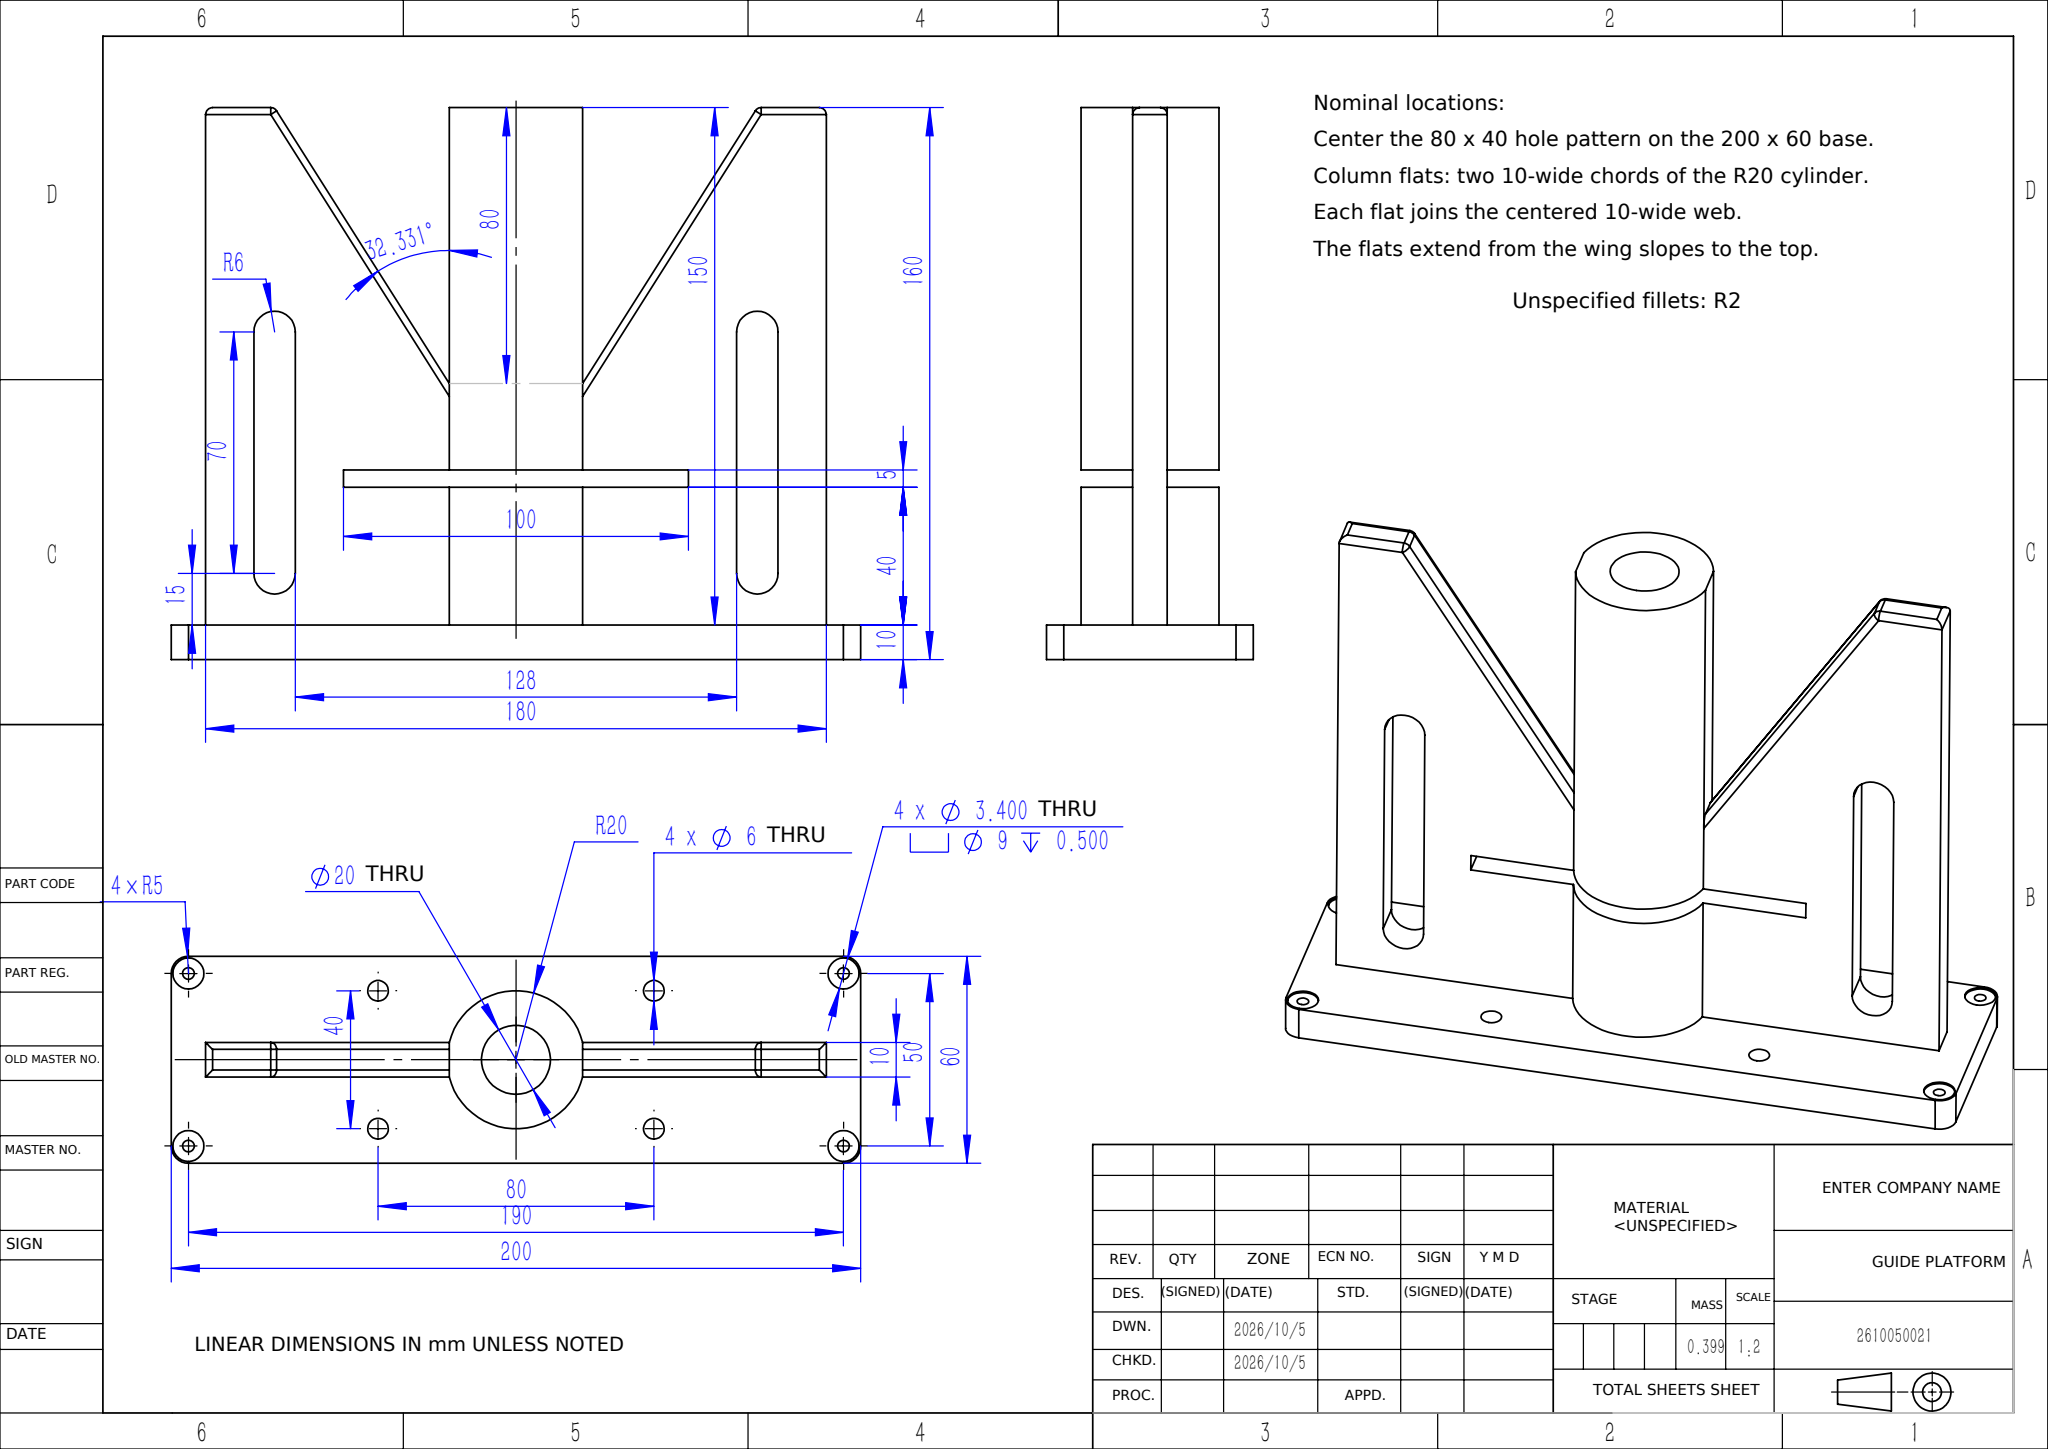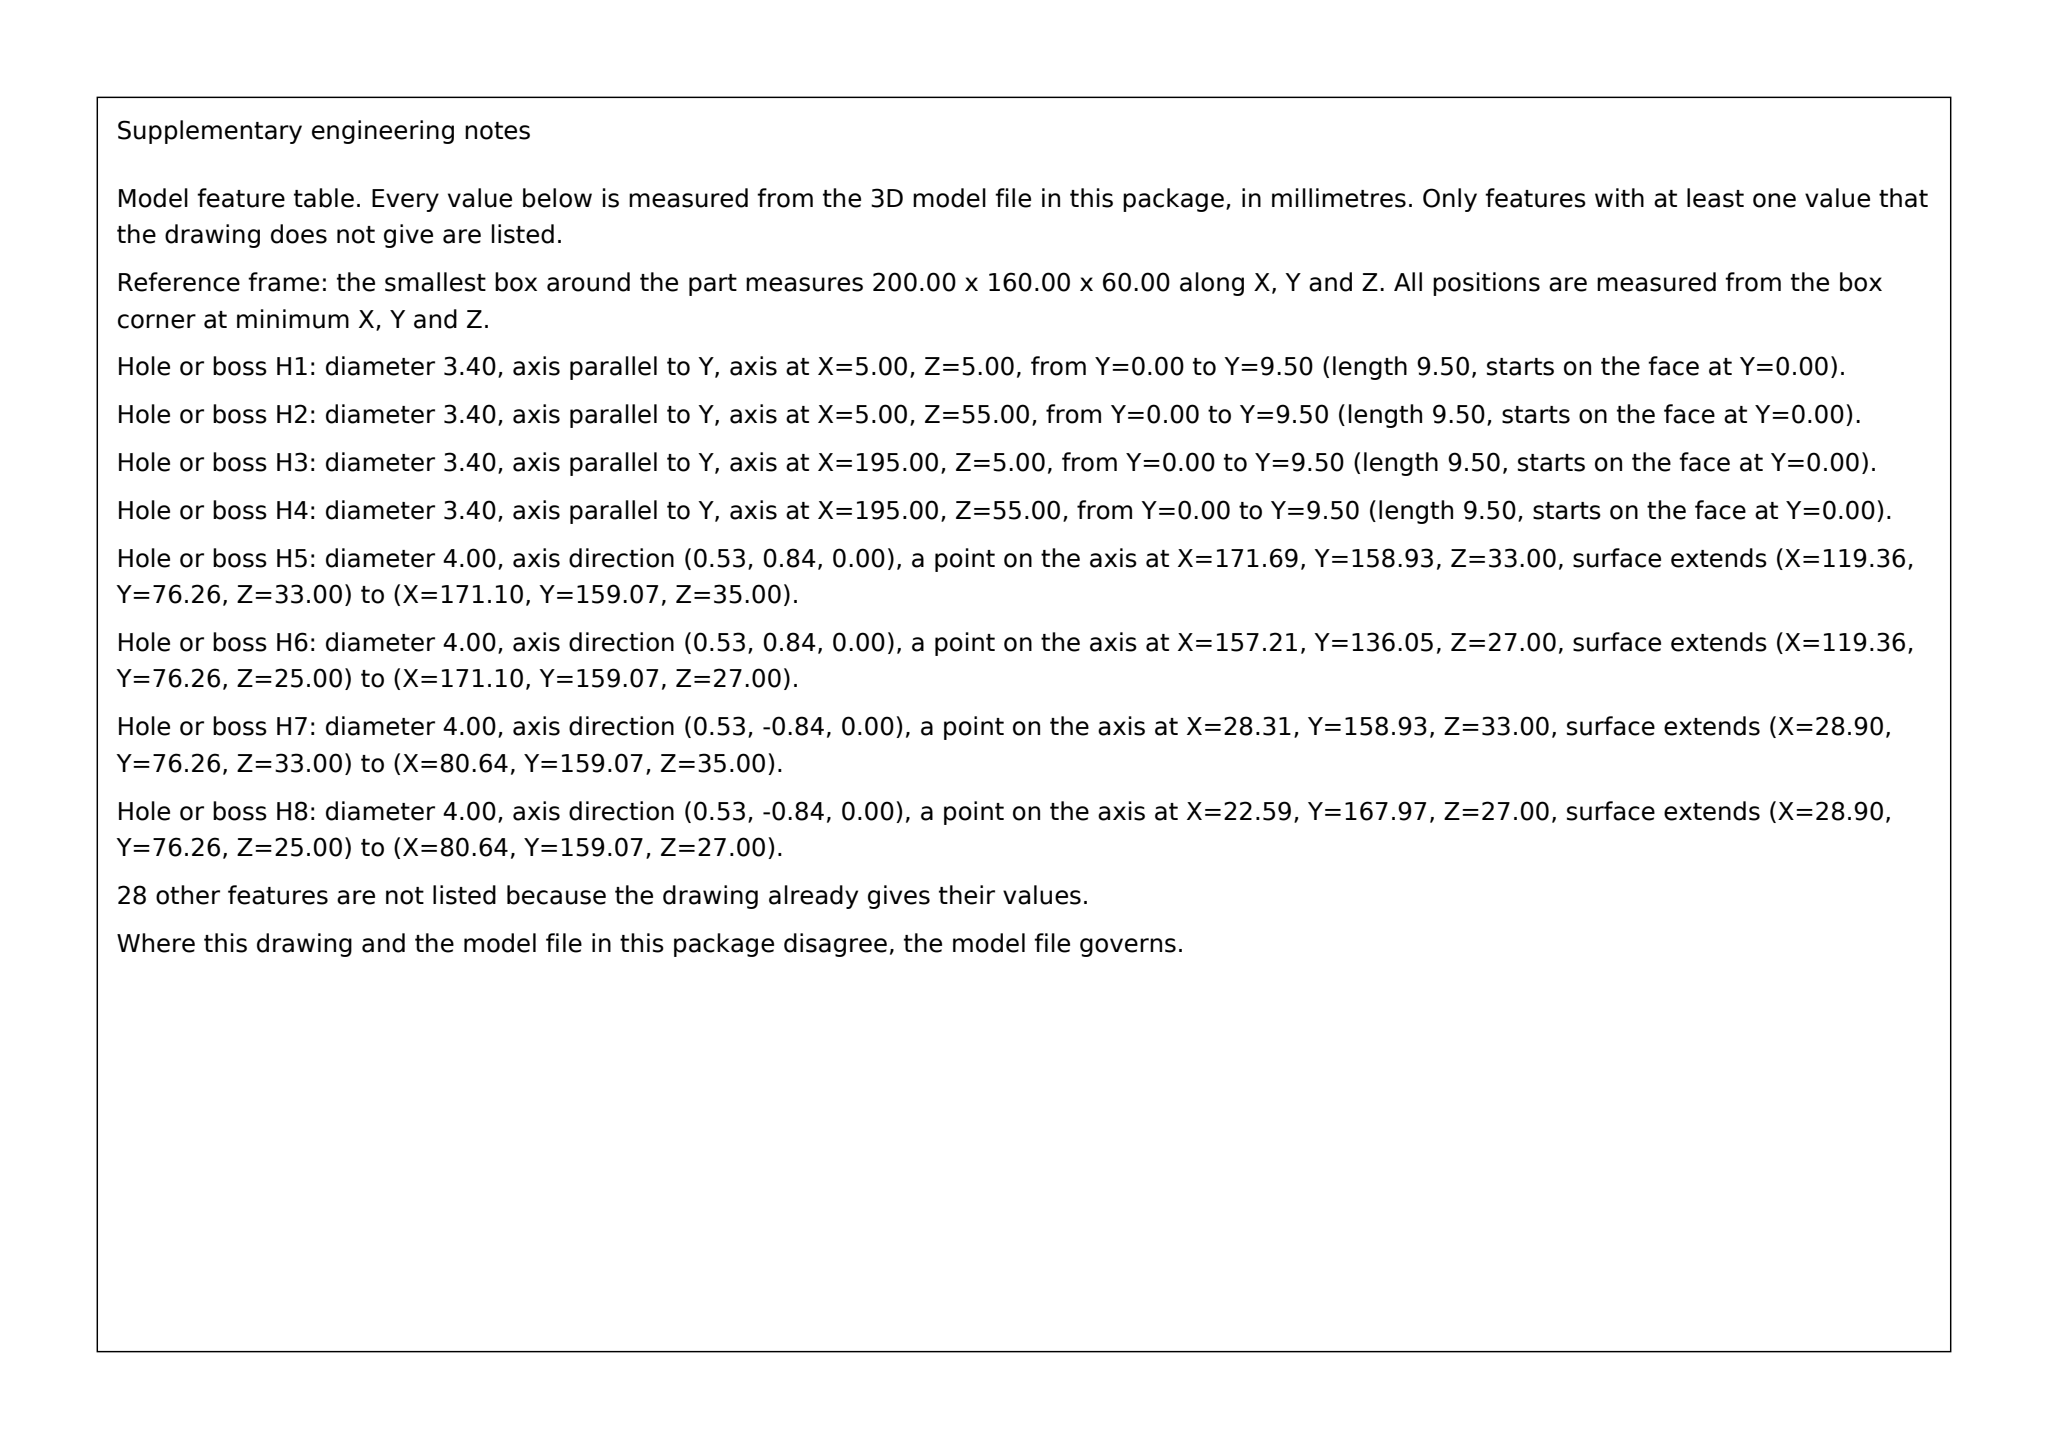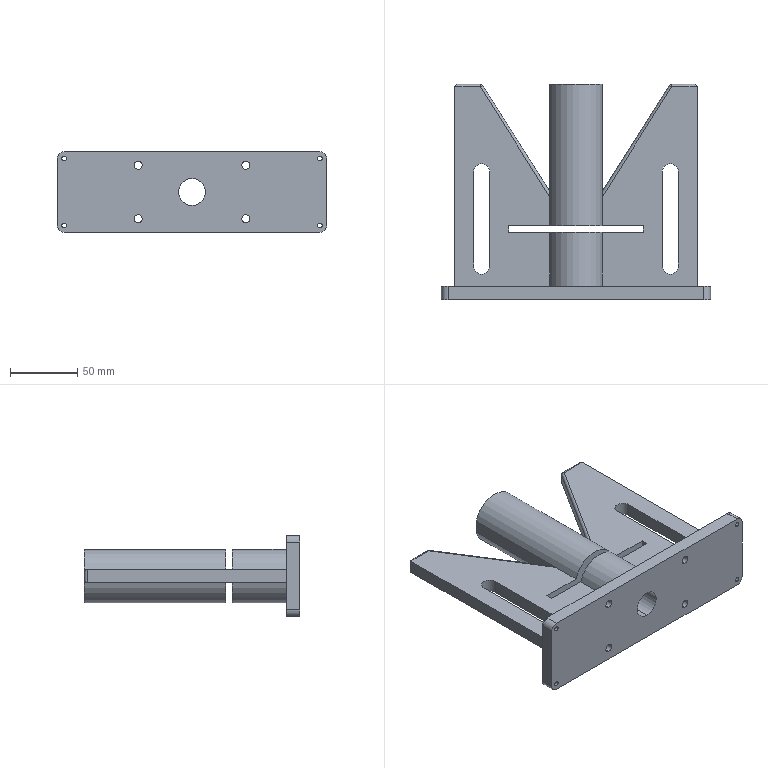Part | SolidWorks | mm | 1 solid | 89 faces | box 200 x 160 x 60 mm | volume 399328 mm3 | cylinder 54 | plane 31 | sphere 4 | commonest cylinder face diameters 4 x12 6 x8 9 x8 3.4 x8 40 x6 20 x4 10 x4 12 x4